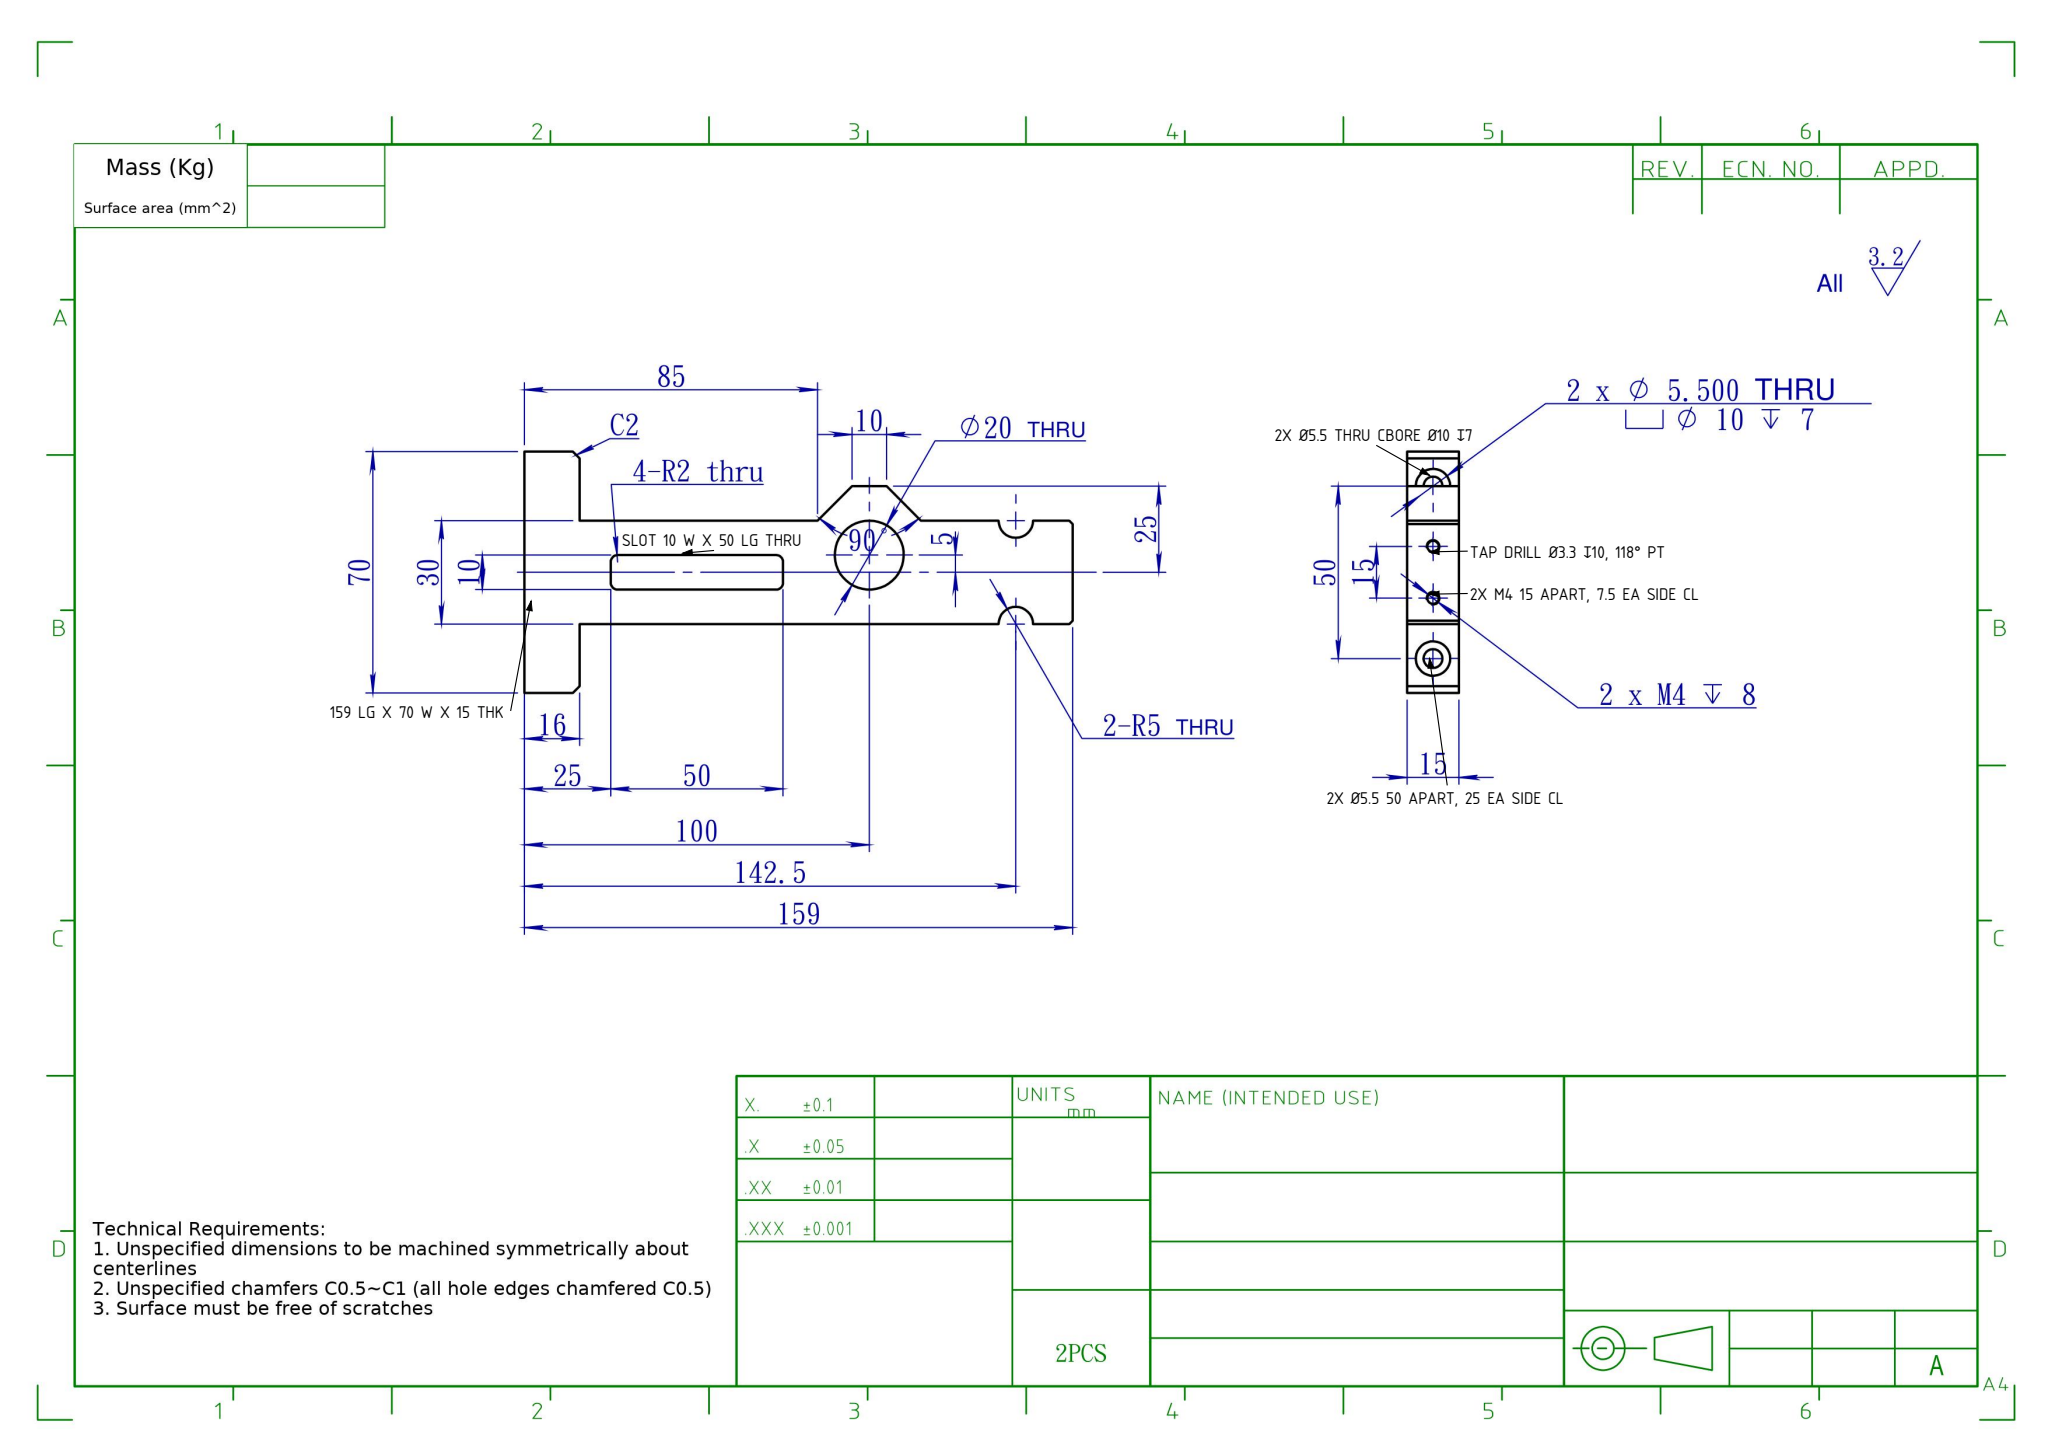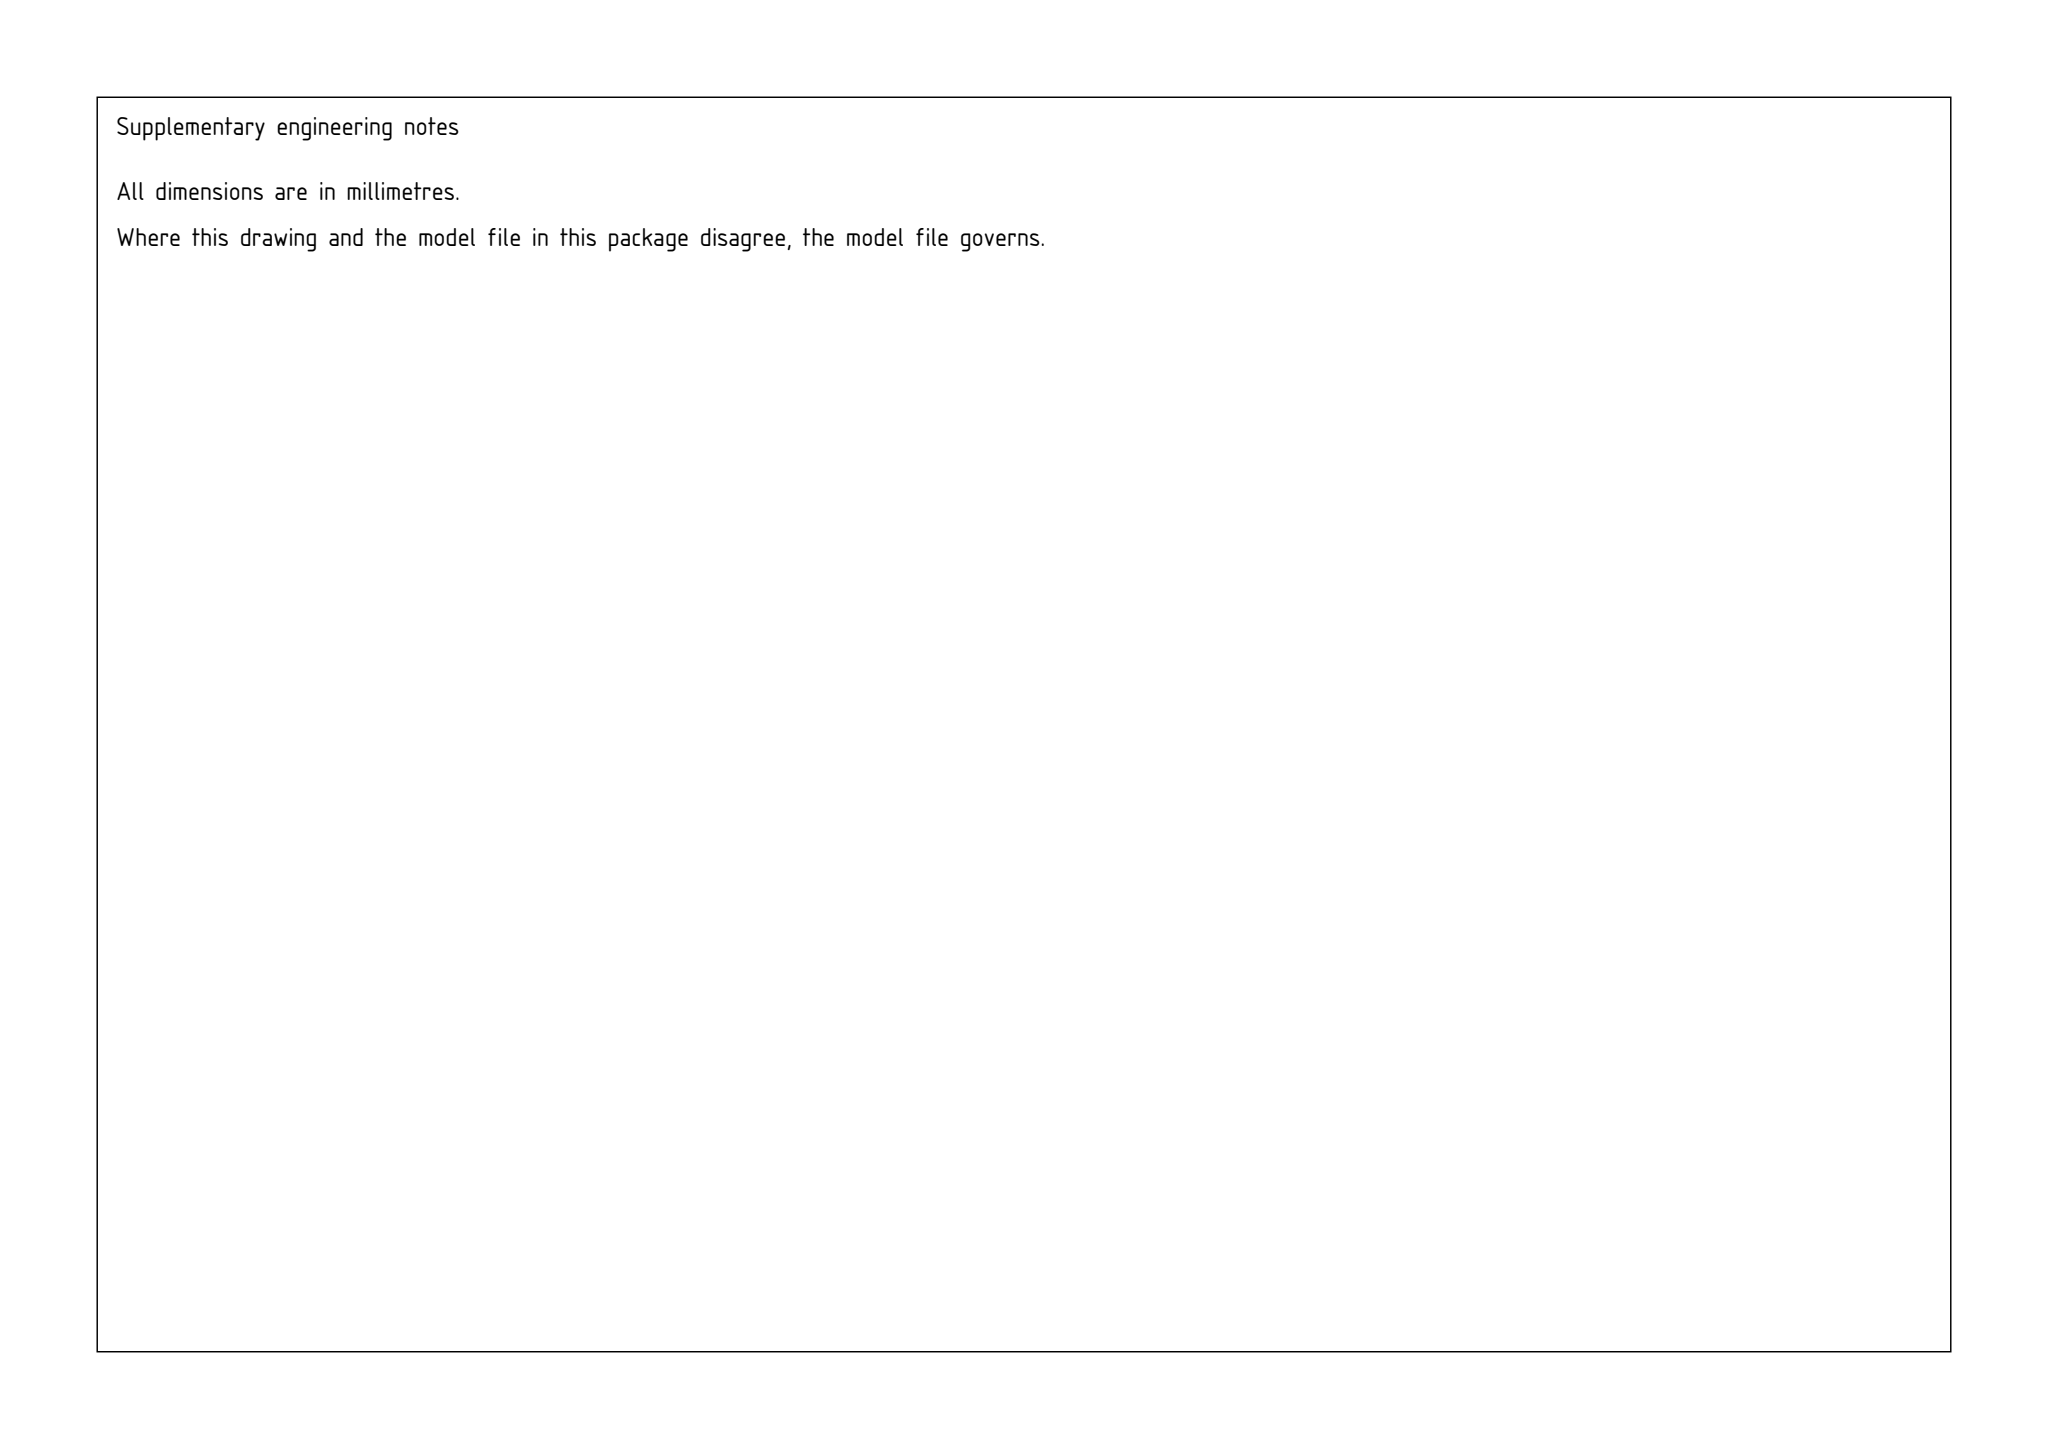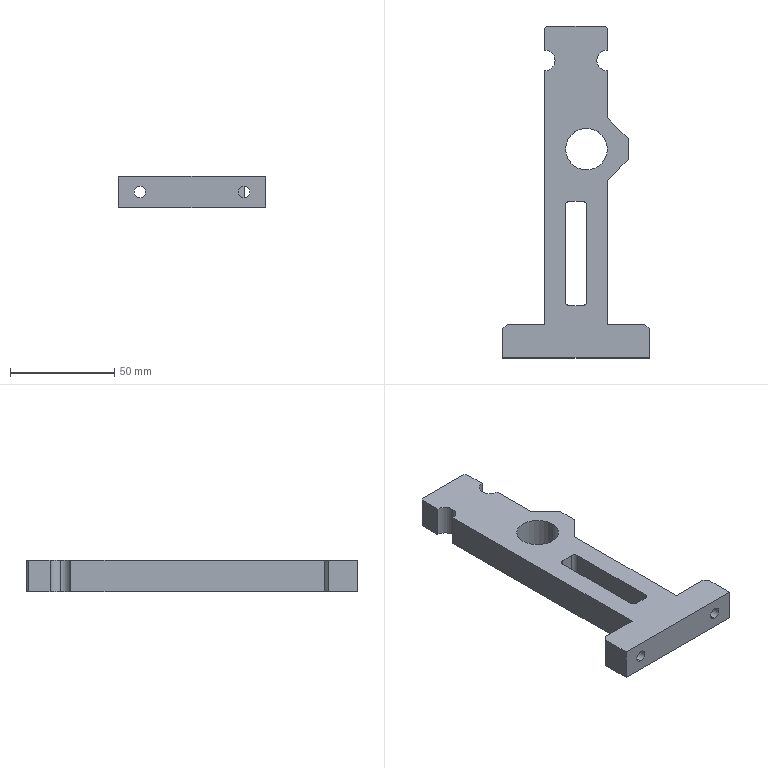Part | SolidWorks | mm | 1 solid | 51 faces | box 70 x 159 x 15 mm | volume 69030 mm3 | plane 26 | cylinder 21 | cone 4 | commonest cylinder face diameters 10 x7 3.3 x4 5.5 x4 4 x4 20 x2
Drawing notes:
STOCK 70 W x 159 LG x 15 THK; FLANGE 16 LG, BODY 50 W SYM ABT CL | from the solid: bbox 70x159x15; y-planes 0/16 flange; x-planes 0/70 flange, 20/50 body; CL x=35
SLOT 10 W x 50 LG THRU 15 THK, 25 TO 75 FROM LH END FACE, 4-R2 CNRS SYM ABT CL | from the solid: x-planes 30/40, y-planes 25/75; R2 (Ø4) cnr cyls axis Z len 15 = full thk, sym abt CL 35
2X Ø5.5 THRU 16 FLANGE, CBORE Ø10 DP 7 FROM LH END FACE, AXES PERP TO IT | from the solid: Ø5.5 axis Y at x=10 & 60, len 9 (y 0-9 side); Ø10 CBORE len 7 from y=0; 7+9=16 flange
2X Ø5.5 CBORE 50 APART, 25 EA SIDE CL, 10 FROM FLANGE EDGE, ON Z CL 7.5 | from the solid: Ø5.5/Ø10 axes at x=10 & 60 in 70 W flange (CL x=35), z=7.5 of 15 thk
2X M4 DP 8 FROM LH END FACE, TAP DRILL Ø3.3 DP 10, 118° PT | from the solid: Ø3.3 cyls axis Y len 10.1 from y=0 face with 118° included-angle cones
2X M4 AXES PERP LH END FACE, ±7.5 FROM CL (15 APART), ON Z CL 7.5 | from the solid: Ø3.3 axis Y at x=27.5 & 42.5 vs CL 35, z=7.5
build123d program:
from build123d import *

# Parameters (mm, degrees)
BOSS_EXTRUDE1_DEPTH                                  = 7.5
COUNTERBORE_FOR_M5_HEX_SOCKET_HEAD_CAP_S_D           = 5.5
COUNTERBORE_FOR_M5_HEX_SOCKET_HEAD_CAP_S_DEPTH       = 16
COUNTERBORE_FOR_M5_HEX_SOCKET_HEAD_CAP_S_CBORE_D     = 10
COUNTERBORE_FOR_M5_HEX_SOCKET_HEAD_CAP_S_CBORE_DEPTH = 7
CHAMFER1_SIZE                                        = 2
CHAMFER2_SIZE                                        = 1
SKETCH7_R                                            = 10
CUT_EXTRUDE2_DEPTH                                   = 148.983
SKETCH8_R                                            = 5
CUT_EXTRUDE3_DEPTH                                   = 148.983
M4_TAPPED_HOLE1_D                                    = 3.3
M4_TAPPED_HOLE1_DEPTH                                = 10.1
M4_TAPPED_HOLE1_TIP                                  = 0.9914


with BuildPart() as part:
    # Sketch1 → Boss-Extrude1 (new, symmetric)
    with BuildSketch(Plane.XY):
        Polygon((-15, 143), (-15, 0), (-35, 0), (-35, -16), (35, -16), (35, 0), (15, 0), (15, 69), (25, 79), (25, 89), (15, 99), (15, 143), align=None)
    extrude(amount=BOSS_EXTRUDE1_DEPTH, both=True)

    # Counterbore for M5 Hex Socket Head Cap S
    with Locations(Plane(origin=(0, 0, 0), x_dir=(1, 0, 0), z_dir=(0, 1, 0))):
        with Locations((-25, 0), (25, 0)):
            CounterBoreHole(COUNTERBORE_FOR_M5_HEX_SOCKET_HEAD_CAP_S_D / 2, COUNTERBORE_FOR_M5_HEX_SOCKET_HEAD_CAP_S_CBORE_D / 2, COUNTERBORE_FOR_M5_HEX_SOCKET_HEAD_CAP_S_CBORE_DEPTH, depth=COUNTERBORE_FOR_M5_HEX_SOCKET_HEAD_CAP_S_DEPTH)

    # Chamfer1
    chamfer1_edges = [part.edges().sort_by_distance(p)[0] for p in [
        (35, 0, 0),
        (-35, 0, 0),
    ]]
    chamfer(chamfer1_edges, length=CHAMFER1_SIZE)

    # Chamfer2
    chamfer2_edges = [part.edges().sort_by_distance(p)[0] for p in [
        (-15, 143, 0),
        (15, 143, 0),
    ]]
    chamfer(chamfer2_edges, length=CHAMFER2_SIZE)

    # Sketch7 → Cut-Extrude2 (cut, through all)
    with BuildSketch(Plane.XY.offset(7.5)):
        with Locations((5, 84)):
            Circle(SKETCH7_R)
        with BuildLine():
            Line((3, 9), (-3, 9))
            ThreePointArc((-3, 9), (-4.414, 9.586), (-5, 11))
            Line((-5, 11), (-5, 57))
            ThreePointArc((-5, 57), (-4.414, 58.414), (-3, 59))
            Line((-3, 59), (3, 59))
            ThreePointArc((3, 59), (4.414, 58.414), (5, 57))
            Line((5, 57), (5, 11))
            ThreePointArc((5, 11), (4.414, 9.586), (3, 9))
        make_face()
    extrude(amount=-CUT_EXTRUDE2_DEPTH, mode=Mode.SUBTRACT)

    # Sketch8 → Cut-Extrude3 (cut, through all)
    with BuildSketch(Plane.XY.offset(7.5)):
        with Locations((-15, 126.5)):
            Circle(SKETCH8_R)
        with Locations((15, 126.5)):
            Circle(SKETCH8_R)
    extrude(amount=-CUT_EXTRUDE3_DEPTH, mode=Mode.SUBTRACT)

    # M4 Tapped Hole1
    with Locations(Plane(origin=(0, 143, 0), x_dir=(1, 0, 0), z_dir=(0, 1, 0))):
        with Locations((-7.5, 0), (7.5, 0)):
            Hole(M4_TAPPED_HOLE1_D / 2, depth=M4_TAPPED_HOLE1_DEPTH)
            with Locations((0, 0, -(M4_TAPPED_HOLE1_DEPTH + M4_TAPPED_HOLE1_TIP / 2))):  # 118° drill point
                Cone(0, M4_TAPPED_HOLE1_D / 2, M4_TAPPED_HOLE1_TIP, mode=Mode.SUBTRACT)


solid = part.part